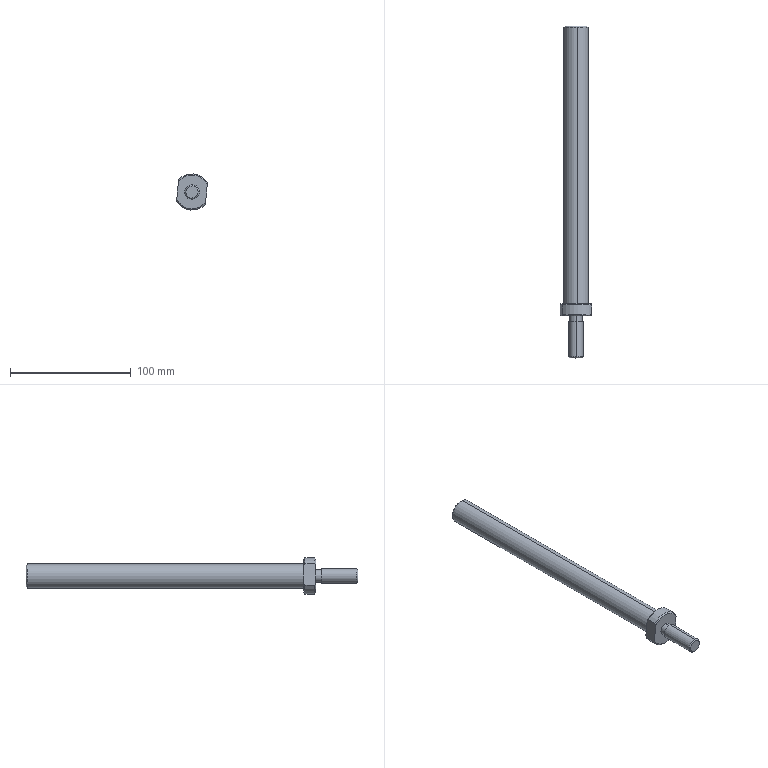Component | SolidWorks | 8TC-A15004-80-16A-3 | 1 solid | 26 faces | box 25.76 x 275 x 30 mm | volume 82271 mm3 | cone 10 | cylinder 9 | plane 7 | commonest cylinder face diameters 30 x3 20 x2 10 x2 12 x2 | material #45
build123d program:
from build123d import *

# Parameters (mm, degrees)
CHAMFER1_SIZE       = 1
SKETCH2_OUTSIDE_W   = 87.65
SKETCH2_OUTSIDE_H   = 87.65
SKETCH2_OUTSIDE_W_2 = 30
SKETCH2_OUTSIDE_H_2 = 24
CUT_EXTRUDE2_DEPTH  = 276.817


with BuildPart() as part:
    # Sketch1 → Revolve3 (revolve)
    with BuildSketch(Plane(origin=(0, 0, 0), x_dir=(1, 0, 0), z_dir=(0, 1, 0)), mode=Mode.PRIVATE) as revolve3_sk:
        Polygon((0, 0), (0, 6), (30, 6), (30, 5), (35, 5), (35, 15), (45, 15), (45, 10), (275, 10), (275, 0), align=None)
    revolve(revolve3_sk.sketch.rotate(Axis((0, 0, 0), (1, 0, 0)), 180), axis=Axis((0, 0, 0), (1, 0, 0)))

    # Chamfer1
    chamfer1_edges = [part.edges().sort_by_distance(p)[0] for p in [
        (0, 0, -6),
        (275, 0, -10),
        (45, 0, -15),
        (35, 0, -15),
    ]]
    chamfer(chamfer1_edges, length=CHAMFER1_SIZE)

    # Sketch2 outside → Cut-Extrude2 (cut, through all)
    with BuildSketch(Plane(origin=(275, 0, 0), x_dir=(0, 0, -1), z_dir=(1, 0, 0))):
        Rectangle(SKETCH2_OUTSIDE_W, SKETCH2_OUTSIDE_H)
        Rectangle(SKETCH2_OUTSIDE_W_2, SKETCH2_OUTSIDE_H_2, mode=Mode.SUBTRACT)
    extrude(amount=-CUT_EXTRUDE2_DEPTH, mode=Mode.SUBTRACT)


solid = part.part

# Placed as in the assembly
solid = solid.moved(Location((40, -42.5, -750), (-180, -6.034, -90)))
STEP:
#1=CARTESIAN_POINT('',(1.554,-1.673,-29.723));
#2=VERTEX_POINT('',#1);
#3=CARTESIAN_POINT('',(1.595,-1.673,-29.332));
#4=VERTEX_POINT('',#3);
#5=CARTESIAN_POINT('',(1.575,-1.673,-29.528));
#6=DIRECTION('',(0.,-1.,0.));
#7=DIRECTION('',(0.1051,0.,0.9945));
#8=AXIS2_PLACEMENT_3D('',#5,#6,#7);
#9=CIRCLE('',#8,0.1969);
#10=EDGE_CURVE('',#2,#4,#9,.T.);
#11=ORIENTED_EDGE('',*,*,#10,.F.);
#12=CARTESIAN_POINT('',(1.55,-1.634,-29.762));
#13=VERTEX_POINT('',#12);
#14=CARTESIAN_POINT('',(1.554,-1.673,-29.723));
#15=DIRECTION('',(-0.07432,0.7071,-0.7032));
#16=VECTOR('',#15,39.37);
#17=LINE('',#14,#16);
#18=EDGE_CURVE('',#2,#13,#17,.T.);
#19=ORIENTED_EDGE('',*,*,#18,.T.);
#20=CARTESIAN_POINT('',(1.6,-1.634,-29.293));
#21=VERTEX_POINT('',#20);
#22=CARTESIAN_POINT('',(1.575,-1.634,-29.528));
#23=DIRECTION('',(0.,1.,0.));
#24=DIRECTION('',(0.1051,0.,0.9945));
#25=AXIS2_PLACEMENT_3D('',#22,#23,#24);
#26=CIRCLE('',#25,0.2362);
#27=EDGE_CURVE('',#21,#13,#26,.T.);
#28=ORIENTED_EDGE('',*,*,#27,.F.);
#29=CARTESIAN_POINT('',(1.595,-1.673,-29.332));
#30=DIRECTION('',(0.07432,0.7071,0.7032));
#31=VECTOR('',#30,39.37);
#32=LINE('',#29,#31);
#33=EDGE_CURVE('',#4,#21,#32,.T.);
#34=ORIENTED_EDGE('',*,*,#33,.F.);
#35=EDGE_LOOP('',(#11,#19,#28,#34));
#36=FACE_OUTER_BOUND('',#35,.T.);
#37=CARTESIAN_POINT('',(1.575,-1.673,-29.528));
#38=DIRECTION('',(0.,1.,0.));
#39=DIRECTION('',(0.1051,0.,0.9945));
#40=AXIS2_PLACEMENT_3D('',#37,#38,#39);
#41=CONICAL_SURFACE('',#40,0.1969,0.7854);
#42=ADVANCED_FACE('',(#36),#41,.T.);
#43=CARTESIAN_POINT('',(1.612,9.154,-29.175));
#44=VERTEX_POINT('',#43);
#45=CARTESIAN_POINT('',(1.538,9.154,-29.88));
#46=VERTEX_POINT('',#45);
#47=CARTESIAN_POINT('',(1.575,9.154,-29.528));
#48=DIRECTION('',(0.,1.,0.));
#49=DIRECTION('',(-0.1051,0.,-0.9945));
#50=AXIS2_PLACEMENT_3D('',#47,#48,#49);
#51=CIRCLE('',#50,0.3543);
#52=EDGE_CURVE('',#44,#46,#51,.T.);
#53=ORIENTED_EDGE('',*,*,#52,.F.);
#54=CARTESIAN_POINT('',(1.616,9.114,-29.136));
#55=VERTEX_POINT('',#54);
#56=CARTESIAN_POINT('',(1.616,9.114,-29.136));
#57=DIRECTION('',(0.07432,-0.7071,0.7032));
#58=VECTOR('',#57,39.37);
#59=LINE('',#56,#58);
#60=EDGE_CURVE('',#44,#55,#59,.T.);
#61=ORIENTED_EDGE('',*,*,#60,.T.);
#62=CARTESIAN_POINT('',(1.533,9.114,-29.919));
#63=VERTEX_POINT('',#62);
#64=CARTESIAN_POINT('',(1.575,9.114,-29.528));
#65=DIRECTION('',(0.,-1.,0.));
#66=DIRECTION('',(-0.1051,0.,-0.9945));
#67=AXIS2_PLACEMENT_3D('',#64,#65,#66);
#68=CIRCLE('',#67,0.3937);
#69=EDGE_CURVE('',#63,#55,#68,.T.);
#70=ORIENTED_EDGE('',*,*,#69,.F.);
#71=CARTESIAN_POINT('',(1.533,9.114,-29.919));
#72=DIRECTION('',(-0.07432,-0.7071,-0.7032));
#73=VECTOR('',#72,39.37);
#74=LINE('',#71,#73);
#75=EDGE_CURVE('',#46,#63,#74,.T.);
#76=ORIENTED_EDGE('',*,*,#75,.F.);
#77=EDGE_LOOP('',(#53,#61,#70,#76));
#78=FACE_OUTER_BOUND('',#77,.T.);
#79=CARTESIAN_POINT('',(1.575,9.114,-29.528));
#80=DIRECTION('',(0.,-1.,0.));
#81=DIRECTION('',(-0.1051,0.,-0.9945));
#82=AXIS2_PLACEMENT_3D('',#79,#80,#81);
#83=CONICAL_SURFACE('',#82,0.3937,0.7854);
#84=ADVANCED_FACE('',(#78),#83,.T.);
#85=ORIENTED_EDGE('',*,*,#69,.T.);
#86=CARTESIAN_POINT('',(1.616,0.09843,-29.136));
#87=VERTEX_POINT('',#86);
#88=CARTESIAN_POINT('',(1.616,-1.673,-29.136));
#89=DIRECTION('',(0.,-1.,0.));
#90=VECTOR('',#89,39.37);
#91=LINE('',#88,#90);
#92=EDGE_CURVE('',#55,#87,#91,.T.);
#93=ORIENTED_EDGE('',*,*,#92,.T.);
#94=CARTESIAN_POINT('',(1.533,0.09843,-29.919));
#95=VERTEX_POINT('',#94);
#96=CARTESIAN_POINT('',(1.575,0.09843,-29.528));
#97=DIRECTION('',(0.,-1.,0.));
#98=DIRECTION('',(-0.1051,0.,-0.9945));
#99=AXIS2_PLACEMENT_3D('',#96,#97,#98);
#100=CIRCLE('',#99,0.3937);
#101=EDGE_CURVE('',#95,#87,#100,.T.);
#102=ORIENTED_EDGE('',*,*,#101,.F.);
#103=CARTESIAN_POINT('',(1.533,-1.673,-29.919));
#104=DIRECTION('',(0.,-1.,0.));
#105=VECTOR('',#104,39.37);
#106=LINE('',#103,#105);
#107=EDGE_CURVE('',#63,#95,#106,.T.);
#108=ORIENTED_EDGE('',*,*,#107,.F.);
#109=EDGE_LOOP('',(#85,#93,#102,#108));
#110=FACE_OUTER_BOUND('',#109,.T.);
#111=CARTESIAN_POINT('',(1.575,-1.673,-29.528));
#112=DIRECTION('',(0.,-1.,0.));
#113=DIRECTION('',(-0.1051,0.,-0.9945));
#114=AXIS2_PLACEMENT_3D('',#111,#112,#113);
#115=CYLINDRICAL_SURFACE('',#114,0.3937);
#116=ADVANCED_FACE('',(#110),#115,.T.);
#117=CARTESIAN_POINT('',(1.554,-0.2953,-29.723));
#118=VERTEX_POINT('',#117);
#119=CARTESIAN_POINT('',(1.595,-0.2953,-29.332));
#120=VERTEX_POINT('',#119);
#121=CARTESIAN_POINT('',(1.575,-0.2953,-29.528));
#122=DIRECTION('',(0.,-1.,0.));
#123=DIRECTION('',(-0.1051,0.,-0.9945));
#124=AXIS2_PLACEMENT_3D('',#121,#122,#123);
#125=CIRCLE('',#124,0.1969);
#126=EDGE_CURVE('',#118,#120,#125,.T.);
#127=ORIENTED_EDGE('',*,*,#126,.T.);
#128=CARTESIAN_POINT('',(1.595,-0.4921,-29.332));
#129=VERTEX_POINT('',#128);
#130=CARTESIAN_POINT('',(1.595,-1.673,-29.332));
#131=DIRECTION('',(0.,-1.,0.));
#132=VECTOR('',#131,39.37);
#133=LINE('',#130,#132);
#134=EDGE_CURVE('',#120,#129,#133,.T.);
#135=ORIENTED_EDGE('',*,*,#134,.T.);
#136=CARTESIAN_POINT('',(1.554,-0.4921,-29.723));
#137=VERTEX_POINT('',#136);
#138=CARTESIAN_POINT('',(1.575,-0.4921,-29.528));
#139=DIRECTION('',(0.,-1.,0.));
#140=DIRECTION('',(-0.1051,0.,-0.9945));
#141=AXIS2_PLACEMENT_3D('',#138,#139,#140);
#142=CIRCLE('',#141,0.1969);
#143=EDGE_CURVE('',#137,#129,#142,.T.);
#144=ORIENTED_EDGE('',*,*,#143,.F.);
#145=CARTESIAN_POINT('',(1.554,-1.673,-29.723));
#146=DIRECTION('',(0.,-1.,0.));
#147=VECTOR('',#146,39.37);
#148=LINE('',#145,#147);
#149=EDGE_CURVE('',#118,#137,#148,.T.);
#150=ORIENTED_EDGE('',*,*,#149,.F.);
#151=EDGE_LOOP('',(#127,#135,#144,#150));
#152=FACE_OUTER_BOUND('',#151,.T.);
#153=CARTESIAN_POINT('',(1.575,-1.673,-29.528));
#154=DIRECTION('',(0.,-1.,0.));
#155=DIRECTION('',(-0.1051,0.,-0.9945));
#156=AXIS2_PLACEMENT_3D('',#153,#154,#155);
#157=CYLINDRICAL_SURFACE('',#156,0.1969);
#158=ADVANCED_FACE('',(#152),#157,.T.);
#159=CARTESIAN_POINT('',(1.55,-0.4921,-29.762));
#160=VERTEX_POINT('',#159);
#161=CARTESIAN_POINT('',(1.6,-0.4921,-29.293));
#162=VERTEX_POINT('',#161);
#163=CARTESIAN_POINT('',(1.575,-0.4921,-29.528));
#164=DIRECTION('',(0.,-1.,0.));
#165=DIRECTION('',(-0.1051,0.,-0.9945));
#166=AXIS2_PLACEMENT_3D('',#163,#164,#165);
#167=CIRCLE('',#166,0.2362);
#168=EDGE_CURVE('',#160,#162,#167,.T.);
#169=ORIENTED_EDGE('',*,*,#168,.T.);
#170=CARTESIAN_POINT('',(1.6,-1.673,-29.293));
#171=DIRECTION('',(0.,-1.,0.));
#172=VECTOR('',#171,39.37);
#173=LINE('',#170,#172);
#174=EDGE_CURVE('',#162,#21,#173,.T.);
#175=ORIENTED_EDGE('',*,*,#174,.T.);
#176=ORIENTED_EDGE('',*,*,#27,.T.);
#177=CARTESIAN_POINT('',(1.55,-1.673,-29.762));
#178=DIRECTION('',(0.,-1.,0.));
#179=VECTOR('',#178,39.37);
#180=LINE('',#177,#179);
#181=EDGE_CURVE('',#160,#13,#180,.T.);
#182=ORIENTED_EDGE('',*,*,#181,.F.);
#183=EDGE_LOOP('',(#169,#175,#176,#182));
#184=FACE_OUTER_BOUND('',#183,.T.);
#185=CARTESIAN_POINT('',(1.575,-1.673,-29.528));
#186=DIRECTION('',(0.,-1.,0.));
#187=DIRECTION('',(-0.1051,0.,-0.9945));
#188=AXIS2_PLACEMENT_3D('',#185,#186,#187);
#189=CYLINDRICAL_SURFACE('',#188,0.2362);
#190=ADVANCED_FACE('',(#184),#189,.T.);
#191=CARTESIAN_POINT('',(1.633,-0.2953,-28.979));
#192=VERTEX_POINT('',#191);
#193=CARTESIAN_POINT('',(1.135,-0.2953,-29.196));
#194=VERTEX_POINT('',#193);
#195=CARTESIAN_POINT('',(1.575,-0.2953,-29.528));
#196=DIRECTION('',(0.,-1.,0.));
#197=DIRECTION('',(0.1051,0.,0.9945));
#198=AXIS2_PLACEMENT_3D('',#195,#196,#197);
#199=CIRCLE('',#198,0.5512);
#200=EDGE_CURVE('',#192,#194,#199,.T.);
#201=ORIENTED_EDGE('',*,*,#200,.F.);
#202=CARTESIAN_POINT('',(1.637,-0.2559,-28.94));
#203=VERTEX_POINT('',#202);
#204=CARTESIAN_POINT('',(1.633,-0.2953,-28.979));
#205=DIRECTION('',(0.07432,0.7071,0.7032));
#206=VECTOR('',#205,39.37);
#207=LINE('',#204,#206);
#208=EDGE_CURVE('',#192,#203,#207,.T.);
#209=ORIENTED_EDGE('',*,*,#208,.T.);
#210=CARTESIAN_POINT('',(1.142,-0.2559,-29.126));
#211=VERTEX_POINT('',#210);
#212=CARTESIAN_POINT('',(1.575,-0.2559,-29.528));
#213=DIRECTION('',(0.,1.,0.));
#214=DIRECTION('',(0.1051,0.,0.9945));
#215=AXIS2_PLACEMENT_3D('',#212,#213,#214);
#216=CIRCLE('',#215,0.5906);
#217=EDGE_CURVE('',#211,#203,#216,.T.);
#218=ORIENTED_EDGE('',*,*,#217,.F.);
#219=CARTESIAN_POINT('',(1.142,-0.2559,-29.126));
#220=CARTESIAN_POINT('',(1.14,-0.2698,-29.149));
#221=CARTESIAN_POINT('',(1.137,-0.283,-29.172));
#222=CARTESIAN_POINT('',(1.135,-0.2953,-29.196));
#223=B_SPLINE_CURVE_WITH_KNOTS('',3,(#219,#220,#221,#222),.UNSPECIFIED.,.F.,.F.,(4,4),(0.02828,0.03033),.UNSPECIFIED.);
#224=EDGE_CURVE('',#211,#194,#223,.T.);
#225=ORIENTED_EDGE('',*,*,#224,.T.);
#226=EDGE_LOOP('',(#201,#209,#218,#225));
#227=FACE_OUTER_BOUND('',#226,.T.);
#228=CARTESIAN_POINT('',(1.575,-0.2953,-29.528));
#229=DIRECTION('',(0.,1.,0.));
#230=DIRECTION('',(0.1051,0.,0.9945));
#231=AXIS2_PLACEMENT_3D('',#228,#229,#230);
#232=CONICAL_SURFACE('',#231,0.5512,0.7854);
#233=ADVANCED_FACE('',(#227),#232,.T.);
#234=CARTESIAN_POINT('',(1.517,0.09843,-30.076));
#235=VERTEX_POINT('',#234);
#236=CARTESIAN_POINT('',(1.075,0.09843,-29.76));
#237=VERTEX_POINT('',#236);
#238=CARTESIAN_POINT('',(1.575,0.09843,-29.528));
#239=DIRECTION('',(0.,1.,0.));
#240=DIRECTION('',(-0.1051,0.,-0.9945));
#241=AXIS2_PLACEMENT_3D('',#238,#239,#240);
#242=CIRCLE('',#241,0.5512);
#243=EDGE_CURVE('',#235,#237,#242,.T.);
#244=ORIENTED_EDGE('',*,*,#243,.F.);
#245=CARTESIAN_POINT('',(1.513,0.05906,-30.115));
#246=VERTEX_POINT('',#245);
#247=CARTESIAN_POINT('',(1.513,0.05906,-30.115));
#248=DIRECTION('',(-0.07432,-0.7071,-0.7032));
#249=VECTOR('',#248,39.37);
#250=LINE('',#247,#249);
#251=EDGE_CURVE('',#235,#246,#250,.T.);
#252=ORIENTED_EDGE('',*,*,#251,.T.);
#253=CARTESIAN_POINT('',(1.068,0.05906,-29.83));
#254=VERTEX_POINT('',#253);
#255=CARTESIAN_POINT('',(1.575,0.05906,-29.528));
#256=DIRECTION('',(0.,-1.,0.));
#257=DIRECTION('',(-0.1051,0.,-0.9945));
#258=AXIS2_PLACEMENT_3D('',#255,#256,#257);
#259=CIRCLE('',#258,0.5906);
#260=EDGE_CURVE('',#254,#246,#259,.T.);
#261=ORIENTED_EDGE('',*,*,#260,.F.);
#262=CARTESIAN_POINT('',(1.068,0.05906,-29.83));
#263=CARTESIAN_POINT('',(1.07,0.07292,-29.807));
#264=CARTESIAN_POINT('',(1.073,0.08613,-29.784));
#265=CARTESIAN_POINT('',(1.075,0.09843,-29.76));
#266=B_SPLINE_CURVE_WITH_KNOTS('',3,(#262,#263,#264,#265),.UNSPECIFIED.,.F.,.F.,(4,4),(0.02828,0.03033),.UNSPECIFIED.);
#267=EDGE_CURVE('',#254,#237,#266,.T.);
#268=ORIENTED_EDGE('',*,*,#267,.T.);
#269=EDGE_LOOP('',(#244,#252,#261,#268));
#270=FACE_OUTER_BOUND('',#269,.T.);
#271=CARTESIAN_POINT('',(1.575,0.05906,-29.528));
#272=DIRECTION('',(0.,-1.,0.));
#273=DIRECTION('',(-0.1051,0.,-0.9945));
#274=AXIS2_PLACEMENT_3D('',#271,#272,#273);
#275=CONICAL_SURFACE('',#274,0.5906,0.7854);
#276=ADVANCED_FACE('',(#270),#275,.T.);
#277=ORIENTED_EDGE('',*,*,#260,.T.);
#278=CARTESIAN_POINT('',(1.513,-0.2559,-30.115));
#279=VERTEX_POINT('',#278);
#280=CARTESIAN_POINT('',(1.513,-1.673,-30.115));
#281=DIRECTION('',(0.,-1.,0.));
#282=VECTOR('',#281,39.37);
#283=LINE('',#280,#282);
#284=EDGE_CURVE('',#246,#279,#283,.T.);
#285=ORIENTED_EDGE('',*,*,#284,.T.);
#286=CARTESIAN_POINT('',(1.068,-0.2559,-29.83));
#287=VERTEX_POINT('',#286);
#288=CARTESIAN_POINT('',(1.575,-0.2559,-29.528));
#289=DIRECTION('',(0.,1.,0.));
#290=DIRECTION('',(0.1051,0.,0.9945));
#291=AXIS2_PLACEMENT_3D('',#288,#289,#290);
#292=CIRCLE('',#291,0.5906);
#293=EDGE_CURVE('',#279,#287,#292,.T.);
#294=ORIENTED_EDGE('',*,*,#293,.T.);
#295=CARTESIAN_POINT('',(1.068,-1.673,-29.83));
#296=DIRECTION('',(0.,-1.,0.));
#297=VECTOR('',#296,39.37);
#298=LINE('',#295,#297);
#299=EDGE_CURVE('',#254,#287,#298,.T.);
#300=ORIENTED_EDGE('',*,*,#299,.F.);
#301=EDGE_LOOP('',(#277,#285,#294,#300));
#302=FACE_OUTER_BOUND('',#301,.T.);
#303=CARTESIAN_POINT('',(1.575,-1.673,-29.528));
#304=DIRECTION('',(0.,-1.,0.));
#305=DIRECTION('',(-0.1051,0.,-0.9945));
#306=AXIS2_PLACEMENT_3D('',#303,#304,#305);
#307=CYLINDRICAL_SURFACE('',#306,0.5906);
#308=ADVANCED_FACE('',(#302),#307,.T.);
#309=ORIENTED_EDGE('',*,*,#126,.F.);
#310=CARTESIAN_POINT('',(1.575,-0.2953,-29.528));
#311=DIRECTION('',(0.,-1.,0.));
#312=DIRECTION('',(-0.1051,0.,-0.9945));
#313=AXIS2_PLACEMENT_3D('',#310,#311,#312);
#314=CIRCLE('',#313,0.1969);
#315=EDGE_CURVE('',#120,#118,#314,.T.);
#316=ORIENTED_EDGE('',*,*,#315,.F.);
#317=EDGE_LOOP('',(#309,#316));
#318=FACE_BOUND('',#317,.T.);
#319=CARTESIAN_POINT('',(1.075,-0.2953,-29.76));
#320=VERTEX_POINT('',#319);
#321=CARTESIAN_POINT('',(1.126,-0.2953,-29.282));
#322=DIRECTION('',(0.1051,0.,0.9945));
#323=VECTOR('',#322,39.37);
#324=LINE('',#321,#323);
#325=EDGE_CURVE('',#320,#194,#324,.T.);
#326=ORIENTED_EDGE('',*,*,#325,.F.);
#327=CARTESIAN_POINT('',(2.015,-0.2953,-29.86));
#328=VERTEX_POINT('',#327);
#329=CARTESIAN_POINT('',(1.575,-0.2953,-29.528));
#330=DIRECTION('',(0.,-1.,0.));
#331=DIRECTION('',(0.1051,0.,0.9945));
#332=AXIS2_PLACEMENT_3D('',#329,#330,#331);
#333=CIRCLE('',#332,0.5512);
#334=EDGE_CURVE('',#320,#328,#333,.T.);
#335=ORIENTED_EDGE('',*,*,#334,.T.);
#336=CARTESIAN_POINT('',(2.074,-0.2953,-29.295));
#337=VERTEX_POINT('',#336);
#338=CARTESIAN_POINT('',(2.065,-0.2953,-29.381));
#339=DIRECTION('',(-0.1051,0.,-0.9945));
#340=VECTOR('',#339,39.37);
#341=LINE('',#338,#340);
#342=EDGE_CURVE('',#337,#328,#341,.T.);
#343=ORIENTED_EDGE('',*,*,#342,.F.);
#344=CARTESIAN_POINT('',(1.575,-0.2953,-29.528));
#345=DIRECTION('',(0.,-1.,0.));
#346=DIRECTION('',(0.1051,0.,0.9945));
#347=AXIS2_PLACEMENT_3D('',#344,#345,#346);
#348=CIRCLE('',#347,0.5512);
#349=EDGE_CURVE('',#337,#192,#348,.T.);
#350=ORIENTED_EDGE('',*,*,#349,.T.);
#351=ORIENTED_EDGE('',*,*,#200,.T.);
#352=EDGE_LOOP('',(#326,#335,#343,#350,#351));
#353=FACE_OUTER_BOUND('',#352,.T.);
#354=CARTESIAN_POINT('',(1.595,-0.2953,-29.332));
#355=DIRECTION('',(0.,1.,0.));
#356=DIRECTION('',(0.1051,0.,0.9945));
#357=AXIS2_PLACEMENT_3D('',#354,#355,#356);
#358=PLANE('',#357);
#359=ADVANCED_FACE('',(#318,#353),#358,.F.);
#360=CARTESIAN_POINT('',(2.082,0.05906,-29.225));
#361=VERTEX_POINT('',#360);
#362=CARTESIAN_POINT('',(1.142,0.05906,-29.126));
#363=VERTEX_POINT('',#362);
#364=CARTESIAN_POINT('',(1.575,0.05906,-29.528));
#365=DIRECTION('',(0.,-1.,0.));
#366=DIRECTION('',(-0.1051,0.,-0.9945));
#367=AXIS2_PLACEMENT_3D('',#364,#365,#366);
#368=CIRCLE('',#367,0.5906);
#369=EDGE_CURVE('',#361,#363,#368,.T.);
#370=ORIENTED_EDGE('',*,*,#369,.T.);
#371=CARTESIAN_POINT('',(1.142,-1.673,-29.126));
#372=DIRECTION('',(0.,1.,0.));
#373=VECTOR('',#372,39.37);
#374=LINE('',#371,#373);
#375=EDGE_CURVE('',#211,#363,#374,.T.);
#376=ORIENTED_EDGE('',*,*,#375,.F.);
#377=ORIENTED_EDGE('',*,*,#217,.T.);
#378=CARTESIAN_POINT('',(2.082,-0.2559,-29.225));
#379=VERTEX_POINT('',#378);
#380=CARTESIAN_POINT('',(1.575,-0.2559,-29.528));
#381=DIRECTION('',(0.,1.,0.));
#382=DIRECTION('',(0.1051,0.,0.9945));
#383=AXIS2_PLACEMENT_3D('',#380,#381,#382);
#384=CIRCLE('',#383,0.5906);
#385=EDGE_CURVE('',#203,#379,#384,.T.);
#386=ORIENTED_EDGE('',*,*,#385,.T.);
#387=CARTESIAN_POINT('',(2.082,-1.673,-29.225));
#388=DIRECTION('',(0.,-1.,0.));
#389=VECTOR('',#388,39.37);
#390=LINE('',#387,#389);
#391=EDGE_CURVE('',#361,#379,#390,.T.);
#392=ORIENTED_EDGE('',*,*,#391,.F.);
#393=EDGE_LOOP('',(#370,#376,#377,#386,#392));
#394=FACE_OUTER_BOUND('',#393,.T.);
#395=CARTESIAN_POINT('',(1.575,-1.673,-29.528));
#396=DIRECTION('',(0.,-1.,0.));
#397=DIRECTION('',(-0.1051,0.,-0.9945));
#398=AXIS2_PLACEMENT_3D('',#395,#396,#397);
#399=CYLINDRICAL_SURFACE('',#398,0.5906);
#400=ADVANCED_FACE('',(#394),#399,.T.);
#401=ORIENTED_EDGE('',*,*,#284,.F.);
#402=CARTESIAN_POINT('',(2.007,0.05906,-29.93));
#403=VERTEX_POINT('',#402);
#404=CARTESIAN_POINT('',(1.575,0.05906,-29.528));
#405=DIRECTION('',(0.,-1.,0.));
#406=DIRECTION('',(-0.1051,0.,-0.9945));
#407=AXIS2_PLACEMENT_3D('',#404,#405,#406);
#408=CIRCLE('',#407,0.5906);
#409=EDGE_CURVE('',#246,#403,#408,.T.);
#410=ORIENTED_EDGE('',*,*,#409,.T.);
#411=CARTESIAN_POINT('',(2.007,-0.2559,-29.93));
#412=VERTEX_POINT('',#411);
#413=CARTESIAN_POINT('',(2.007,-1.673,-29.93));
#414=DIRECTION('',(0.,1.,0.));
#415=VECTOR('',#414,39.37);
#416=LINE('',#413,#415);
#417=EDGE_CURVE('',#412,#403,#416,.T.);
#418=ORIENTED_EDGE('',*,*,#417,.F.);
#419=CARTESIAN_POINT('',(1.575,-0.2559,-29.528));
#420=DIRECTION('',(0.,1.,0.));
#421=DIRECTION('',(0.1051,0.,0.9945));
#422=AXIS2_PLACEMENT_3D('',#419,#420,#421);
#423=CIRCLE('',#422,0.5906);
#424=EDGE_CURVE('',#412,#279,#423,.T.);
#425=ORIENTED_EDGE('',*,*,#424,.T.);
#426=EDGE_LOOP('',(#401,#410,#418,#425));
#427=FACE_OUTER_BOUND('',#426,.T.);
#428=CARTESIAN_POINT('',(1.575,-1.673,-29.528));
#429=DIRECTION('',(0.,-1.,0.));
#430=DIRECTION('',(-0.1051,0.,-0.9945));
#431=AXIS2_PLACEMENT_3D('',#428,#429,#430);
#432=CYLINDRICAL_SURFACE('',#431,0.5906);
#433=ADVANCED_FACE('',(#427),#432,.T.);
#434=ORIENTED_EDGE('',*,*,#101,.T.);
#435=CARTESIAN_POINT('',(1.575,0.09843,-29.528));
#436=DIRECTION('',(0.,-1.,0.));
#437=DIRECTION('',(-0.1051,0.,-0.9945));
#438=AXIS2_PLACEMENT_3D('',#435,#436,#437);
#439=CIRCLE('',#438,0.3937);
#440=EDGE_CURVE('',#87,#95,#439,.T.);
#441=ORIENTED_EDGE('',*,*,#440,.T.);
#442=EDGE_LOOP('',(#434,#441));
#443=FACE_BOUND('',#442,.T.);
#444=CARTESIAN_POINT('',(1.135,0.09843,-29.196));
#445=VERTEX_POINT('',#444);
#446=CARTESIAN_POINT('',(1.167,0.09843,-28.891));
#447=DIRECTION('',(-0.1051,0.,-0.9945));
#448=VECTOR('',#447,39.37);
#449=LINE('',#446,#448);
#450=EDGE_CURVE('',#445,#237,#449,.T.);
#451=ORIENTED_EDGE('',*,*,#450,.F.);
#452=CARTESIAN_POINT('',(2.074,0.09843,-29.295));
#453=VERTEX_POINT('',#452);
#454=CARTESIAN_POINT('',(1.575,0.09843,-29.528));
#455=DIRECTION('',(0.,1.,0.));
#456=DIRECTION('',(-0.1051,0.,-0.9945));
#457=AXIS2_PLACEMENT_3D('',#454,#455,#456);
#458=CIRCLE('',#457,0.5512);
#459=EDGE_CURVE('',#445,#453,#458,.T.);
#460=ORIENTED_EDGE('',*,*,#459,.T.);
#461=CARTESIAN_POINT('',(2.015,0.09843,-29.86));
#462=VERTEX_POINT('',#461);
#463=CARTESIAN_POINT('',(2.107,0.09843,-28.99));
#464=DIRECTION('',(0.1051,0.,0.9945));
#465=VECTOR('',#464,39.37);
#466=LINE('',#463,#465);
#467=EDGE_CURVE('',#462,#453,#466,.T.);
#468=ORIENTED_EDGE('',*,*,#467,.F.);
#469=CARTESIAN_POINT('',(1.575,0.09843,-29.528));
#470=DIRECTION('',(0.,1.,0.));
#471=DIRECTION('',(-0.1051,0.,-0.9945));
#472=AXIS2_PLACEMENT_3D('',#469,#470,#471);
#473=CIRCLE('',#472,0.5512);
#474=EDGE_CURVE('',#462,#235,#473,.T.);
#475=ORIENTED_EDGE('',*,*,#474,.T.);
#476=ORIENTED_EDGE('',*,*,#243,.T.);
#477=EDGE_LOOP('',(#451,#460,#468,#475,#476));
#478=FACE_OUTER_BOUND('',#477,.T.);
#479=CARTESIAN_POINT('',(1.637,0.09843,-28.94));
#480=DIRECTION('',(0.,-1.,0.));
#481=DIRECTION('',(-0.1051,0.,-0.9945));
#482=AXIS2_PLACEMENT_3D('',#479,#480,#481);
#483=PLANE('',#482);
#484=ADVANCED_FACE('',(#443,#478),#483,.F.);
#485=ORIENTED_EDGE('',*,*,#251,.F.);
#486=ORIENTED_EDGE('',*,*,#474,.F.);
#487=CARTESIAN_POINT('',(2.015,0.09843,-29.86));
#488=CARTESIAN_POINT('',(2.012,0.0861,-29.883));
#489=CARTESIAN_POINT('',(2.01,0.0729,-29.907));
#490=CARTESIAN_POINT('',(2.007,0.05906,-29.93));
#491=B_SPLINE_CURVE_WITH_KNOTS('',3,(#487,#488,#489,#490),.UNSPECIFIED.,.F.,.F.,(4,4),(0.04546,0.04753),.UNSPECIFIED.);
#492=EDGE_CURVE('',#462,#403,#491,.T.);
#493=ORIENTED_EDGE('',*,*,#492,.T.);
#494=ORIENTED_EDGE('',*,*,#409,.F.);
#495=EDGE_LOOP('',(#485,#486,#493,#494));
#496=FACE_OUTER_BOUND('',#495,.T.);
#497=CARTESIAN_POINT('',(1.575,0.05906,-29.528));
#498=DIRECTION('',(0.,-1.,0.));
#499=DIRECTION('',(-0.1051,0.,-0.9945));
#500=AXIS2_PLACEMENT_3D('',#497,#498,#499);
#501=CONICAL_SURFACE('',#500,0.5906,0.7854);
#502=ADVANCED_FACE('',(#496),#501,.T.);
#503=ORIENTED_EDGE('',*,*,#459,.F.);
#504=CARTESIAN_POINT('',(1.135,0.09843,-29.196));
#505=CARTESIAN_POINT('',(1.137,0.0861,-29.172));
#506=CARTESIAN_POINT('',(1.14,0.0729,-29.148));
#507=CARTESIAN_POINT('',(1.142,0.05906,-29.126));
#508=B_SPLINE_CURVE_WITH_KNOTS('',3,(#504,#505,#506,#507),.UNSPECIFIED.,.F.,.F.,(4,4),(0.04546,0.04753),.UNSPECIFIED.);
#509=EDGE_CURVE('',#445,#363,#508,.T.);
#510=ORIENTED_EDGE('',*,*,#509,.T.);
#511=ORIENTED_EDGE('',*,*,#369,.F.);
#512=CARTESIAN_POINT('',(2.082,0.05906,-29.225));
#513=CARTESIAN_POINT('',(2.079,0.07292,-29.248));
#514=CARTESIAN_POINT('',(2.077,0.08613,-29.271));
#515=CARTESIAN_POINT('',(2.074,0.09843,-29.295));
#516=B_SPLINE_CURVE_WITH_KNOTS('',3,(#512,#513,#514,#515),.UNSPECIFIED.,.F.,.F.,(4,4),(0.02828,0.03033),.UNSPECIFIED.);
#517=EDGE_CURVE('',#361,#453,#516,.T.);
#518=ORIENTED_EDGE('',*,*,#517,.T.);
#519=EDGE_LOOP('',(#503,#510,#511,#518));
#520=FACE_OUTER_BOUND('',#519,.T.);
#521=CARTESIAN_POINT('',(1.575,0.05906,-29.528));
#522=DIRECTION('',(0.,-1.,0.));
#523=DIRECTION('',(-0.1051,0.,-0.9945));
#524=AXIS2_PLACEMENT_3D('',#521,#522,#523);
#525=CONICAL_SURFACE('',#524,0.5906,0.7854);
#526=ADVANCED_FACE('',(#520),#525,.T.);
#527=ORIENTED_EDGE('',*,*,#208,.F.);
#528=ORIENTED_EDGE('',*,*,#349,.F.);
#529=CARTESIAN_POINT('',(2.074,-0.2953,-29.295));
#530=CARTESIAN_POINT('',(2.077,-0.2829,-29.271));
#531=CARTESIAN_POINT('',(2.079,-0.2697,-29.248));
#532=CARTESIAN_POINT('',(2.082,-0.2559,-29.225));
#533=B_SPLINE_CURVE_WITH_KNOTS('',3,(#529,#530,#531,#532),.UNSPECIFIED.,.F.,.F.,(4,4),(0.04546,0.04753),.UNSPECIFIED.);
#534=EDGE_CURVE('',#337,#379,#533,.T.);
#535=ORIENTED_EDGE('',*,*,#534,.T.);
#536=ORIENTED_EDGE('',*,*,#385,.F.);
#537=EDGE_LOOP('',(#527,#528,#535,#536));
#538=FACE_OUTER_BOUND('',#537,.T.);
#539=CARTESIAN_POINT('',(1.575,-0.2953,-29.528));
#540=DIRECTION('',(0.,1.,0.));
#541=DIRECTION('',(0.1051,0.,0.9945));
#542=AXIS2_PLACEMENT_3D('',#539,#540,#541);
#543=CONICAL_SURFACE('',#542,0.5512,0.7854);
#544=ADVANCED_FACE('',(#538),#543,.T.);
#545=ORIENTED_EDGE('',*,*,#334,.F.);
#546=CARTESIAN_POINT('',(1.075,-0.2953,-29.76));
#547=CARTESIAN_POINT('',(1.073,-0.2829,-29.784));
#548=CARTESIAN_POINT('',(1.07,-0.2697,-29.807));
#549=CARTESIAN_POINT('',(1.068,-0.2559,-29.83));
#550=B_SPLINE_CURVE_WITH_KNOTS('',3,(#546,#547,#548,#549),.UNSPECIFIED.,.F.,.F.,(4,4),(0.04546,0.04753),.UNSPECIFIED.);
#551=EDGE_CURVE('',#320,#287,#550,.T.);
#552=ORIENTED_EDGE('',*,*,#551,.T.);
#553=ORIENTED_EDGE('',*,*,#293,.F.);
#554=ORIENTED_EDGE('',*,*,#424,.F.);
#555=CARTESIAN_POINT('',(2.007,-0.2559,-29.93));
#556=CARTESIAN_POINT('',(2.01,-0.2698,-29.907));
#557=CARTESIAN_POINT('',(2.012,-0.283,-29.883));
#558=CARTESIAN_POINT('',(2.015,-0.2953,-29.86));
#559=B_SPLINE_CURVE_WITH_KNOTS('',3,(#555,#556,#557,#558),.UNSPECIFIED.,.F.,.F.,(4,4),(0.02828,0.03033),.UNSPECIFIED.);
#560=EDGE_CURVE('',#412,#328,#559,.T.);
#561=ORIENTED_EDGE('',*,*,#560,.T.);
#562=EDGE_LOOP('',(#545,#552,#553,#554,#561));
#563=FACE_OUTER_BOUND('',#562,.T.);
#564=CARTESIAN_POINT('',(1.575,-0.2953,-29.528));
#565=DIRECTION('',(0.,1.,0.));
#566=DIRECTION('',(0.1051,0.,0.9945));
#567=AXIS2_PLACEMENT_3D('',#564,#565,#566);
#568=CONICAL_SURFACE('',#567,0.5512,0.7854);
#569=ADVANCED_FACE('',(#563),#568,.T.);
#570=CARTESIAN_POINT('',(1.575,-1.673,-29.528));
#571=DIRECTION('',(0.,-1.,0.));
#572=DIRECTION('',(0.1051,0.,0.9945));
#573=AXIS2_PLACEMENT_3D('',#570,#571,#572);
#574=CIRCLE('',#573,0.1969);
#575=EDGE_CURVE('',#4,#2,#574,.T.);
#576=ORIENTED_EDGE('',*,*,#575,.T.);
#577=ORIENTED_EDGE('',*,*,#10,.T.);
#578=EDGE_LOOP('',(#576,#577));
#579=FACE_OUTER_BOUND('',#578,.T.);
#580=CARTESIAN_POINT('',(1.575,-1.673,-29.528));
#581=DIRECTION('',(0.,1.,0.));
#582=DIRECTION('',(0.1051,0.,0.9945));
#583=AXIS2_PLACEMENT_3D('',#580,#581,#582);
#584=PLANE('',#583);
#585=ADVANCED_FACE('',(#579),#584,.F.);
#586=ORIENTED_EDGE('',*,*,#174,.F.);
#587=CARTESIAN_POINT('',(1.575,-0.4921,-29.528));
#588=DIRECTION('',(0.,-1.,0.));
#589=DIRECTION('',(-0.1051,0.,-0.9945));
#590=AXIS2_PLACEMENT_3D('',#587,#588,#589);
#591=CIRCLE('',#590,0.2362);
#592=EDGE_CURVE('',#162,#160,#591,.T.);
#593=ORIENTED_EDGE('',*,*,#592,.T.);
#594=ORIENTED_EDGE('',*,*,#181,.T.);
#595=CARTESIAN_POINT('',(1.575,-1.634,-29.528));
#596=DIRECTION('',(0.,1.,0.));
#597=DIRECTION('',(0.1051,0.,0.9945));
#598=AXIS2_PLACEMENT_3D('',#595,#596,#597);
#599=CIRCLE('',#598,0.2362);
#600=EDGE_CURVE('',#13,#21,#599,.T.);
#601=ORIENTED_EDGE('',*,*,#600,.T.);
#602=EDGE_LOOP('',(#586,#593,#594,#601));
#603=FACE_OUTER_BOUND('',#602,.T.);
#604=CARTESIAN_POINT('',(1.575,-1.673,-29.528));
#605=DIRECTION('',(0.,-1.,0.));
#606=DIRECTION('',(-0.1051,0.,-0.9945));
#607=AXIS2_PLACEMENT_3D('',#604,#605,#606);
#608=CYLINDRICAL_SURFACE('',#607,0.2362);
#609=ADVANCED_FACE('',(#603),#608,.T.);
#610=ORIENTED_EDGE('',*,*,#168,.F.);
#611=ORIENTED_EDGE('',*,*,#592,.F.);
#612=EDGE_LOOP('',(#610,#611));
#613=FACE_OUTER_BOUND('',#612,.T.);
#614=ORIENTED_EDGE('',*,*,#143,.T.);
#615=CARTESIAN_POINT('',(1.575,-0.4921,-29.528));
#616=DIRECTION('',(0.,-1.,0.));
#617=DIRECTION('',(-0.1051,0.,-0.9945));
#618=AXIS2_PLACEMENT_3D('',#615,#616,#617);
#619=CIRCLE('',#618,0.1969);
#620=EDGE_CURVE('',#129,#137,#619,.T.);
#621=ORIENTED_EDGE('',*,*,#620,.T.);
#622=EDGE_LOOP('',(#614,#621));
#623=FACE_BOUND('',#622,.T.);
#624=CARTESIAN_POINT('',(1.6,-0.4921,-29.293));
#625=DIRECTION('',(0.,-1.,0.));
#626=DIRECTION('',(-0.1051,0.,-0.9945));
#627=AXIS2_PLACEMENT_3D('',#624,#625,#626);
#628=PLANE('',#627);
#629=ADVANCED_FACE('',(#613,#623),#628,.F.);
#630=ORIENTED_EDGE('',*,*,#134,.F.);
#631=ORIENTED_EDGE('',*,*,#315,.T.);
#632=ORIENTED_EDGE('',*,*,#149,.T.);
#633=ORIENTED_EDGE('',*,*,#620,.F.);
#634=EDGE_LOOP('',(#630,#631,#632,#633));
#635=FACE_OUTER_BOUND('',#634,.T.);
#636=CARTESIAN_POINT('',(1.575,-1.673,-29.528));
#637=DIRECTION('',(0.,-1.,0.));
#638=DIRECTION('',(-0.1051,0.,-0.9945));
#639=AXIS2_PLACEMENT_3D('',#636,#637,#638);
#640=CYLINDRICAL_SURFACE('',#639,0.1969);
#641=ADVANCED_FACE('',(#635),#640,.T.);
#642=ORIENTED_EDGE('',*,*,#92,.F.);
#643=CARTESIAN_POINT('',(1.575,9.114,-29.528));
#644=DIRECTION('',(0.,-1.,0.));
#645=DIRECTION('',(-0.1051,0.,-0.9945));
#646=AXIS2_PLACEMENT_3D('',#643,#644,#645);
#647=CIRCLE('',#646,0.3937);
#648=EDGE_CURVE('',#55,#63,#647,.T.);
#649=ORIENTED_EDGE('',*,*,#648,.T.);
#650=ORIENTED_EDGE('',*,*,#107,.T.);
#651=ORIENTED_EDGE('',*,*,#440,.F.);
#652=EDGE_LOOP('',(#642,#649,#650,#651));
#653=FACE_OUTER_BOUND('',#652,.T.);
#654=CARTESIAN_POINT('',(1.575,-1.673,-29.528));
#655=DIRECTION('',(0.,-1.,0.));
#656=DIRECTION('',(-0.1051,0.,-0.9945));
#657=AXIS2_PLACEMENT_3D('',#654,#655,#656);
#658=CYLINDRICAL_SURFACE('',#657,0.3937);
#659=ADVANCED_FACE('',(#653),#658,.T.);
#660=CARTESIAN_POINT('',(1.575,9.154,-29.528));
#661=DIRECTION('',(0.,1.,0.));
#662=DIRECTION('',(-0.1051,0.,-0.9945));
#663=AXIS2_PLACEMENT_3D('',#660,#661,#662);
#664=CIRCLE('',#663,0.3543);
#665=EDGE_CURVE('',#46,#44,#664,.T.);
#666=ORIENTED_EDGE('',*,*,#665,.T.);
#667=ORIENTED_EDGE('',*,*,#52,.T.);
#668=EDGE_LOOP('',(#666,#667));
#669=FACE_OUTER_BOUND('',#668,.T.);
#670=CARTESIAN_POINT('',(1.616,9.154,-29.136));
#671=DIRECTION('',(0.,-1.,0.));
#672=DIRECTION('',(-0.1051,0.,-0.9945));
#673=AXIS2_PLACEMENT_3D('',#670,#671,#672);
#674=PLANE('',#673);
#675=ADVANCED_FACE('',(#669),#674,.F.);
#676=ORIENTED_EDGE('',*,*,#60,.F.);
#677=ORIENTED_EDGE('',*,*,#665,.F.);
#678=ORIENTED_EDGE('',*,*,#75,.T.);
#679=ORIENTED_EDGE('',*,*,#648,.F.);
#680=EDGE_LOOP('',(#676,#677,#678,#679));
#681=FACE_OUTER_BOUND('',#680,.T.);
#682=CARTESIAN_POINT('',(1.575,9.114,-29.528));
#683=DIRECTION('',(0.,-1.,0.));
#684=DIRECTION('',(-0.1051,0.,-0.9945));
#685=AXIS2_PLACEMENT_3D('',#682,#683,#684);
#686=CONICAL_SURFACE('',#685,0.3937,0.7854);
#687=ADVANCED_FACE('',(#681),#686,.T.);
#688=ORIENTED_EDGE('',*,*,#18,.F.);
#689=ORIENTED_EDGE('',*,*,#575,.F.);
#690=ORIENTED_EDGE('',*,*,#33,.T.);
#691=ORIENTED_EDGE('',*,*,#600,.F.);
#692=EDGE_LOOP('',(#688,#689,#690,#691));
#693=FACE_OUTER_BOUND('',#692,.T.);
#694=CARTESIAN_POINT('',(1.575,-1.673,-29.528));
#695=DIRECTION('',(0.,1.,0.));
#696=DIRECTION('',(0.1051,0.,0.9945));
#697=AXIS2_PLACEMENT_3D('',#694,#695,#696);
#698=CONICAL_SURFACE('',#697,0.1969,0.7854);
#699=ADVANCED_FACE('',(#693),#698,.T.);
#700=ORIENTED_EDGE('',*,*,#467,.T.);
#701=ORIENTED_EDGE('',*,*,#517,.F.);
#702=ORIENTED_EDGE('',*,*,#391,.T.);
#703=ORIENTED_EDGE('',*,*,#534,.F.);
#704=ORIENTED_EDGE('',*,*,#342,.T.);
#705=ORIENTED_EDGE('',*,*,#560,.F.);
#706=ORIENTED_EDGE('',*,*,#417,.T.);
#707=ORIENTED_EDGE('',*,*,#492,.F.);
#708=EDGE_LOOP('',(#700,#701,#702,#703,#704,#705,#706,#707));
#709=FACE_OUTER_BOUND('',#708,.T.);
#710=CARTESIAN_POINT('',(1.983,-1.673,-30.164));
#711=DIRECTION('',(0.9945,0.,-0.1051));
#712=DIRECTION('',(-0.1051,0.,-0.9945));
#713=AXIS2_PLACEMENT_3D('',#710,#711,#712);
#714=PLANE('',#713);
#715=ADVANCED_FACE('',(#709),#714,.T.);
#716=ORIENTED_EDGE('',*,*,#450,.T.);
#717=ORIENTED_EDGE('',*,*,#267,.F.);
#718=ORIENTED_EDGE('',*,*,#299,.T.);
#719=ORIENTED_EDGE('',*,*,#551,.F.);
#720=ORIENTED_EDGE('',*,*,#325,.T.);
#721=ORIENTED_EDGE('',*,*,#224,.F.);
#722=ORIENTED_EDGE('',*,*,#375,.T.);
#723=ORIENTED_EDGE('',*,*,#509,.F.);
#724=EDGE_LOOP('',(#716,#717,#718,#719,#720,#721,#722,#723));
#725=FACE_OUTER_BOUND('',#724,.T.);
#726=CARTESIAN_POINT('',(1.043,-1.673,-30.065));
#727=DIRECTION('',(-0.9945,0.,0.1051));
#728=DIRECTION('',(0.1051,0.,0.9945));
#729=AXIS2_PLACEMENT_3D('',#726,#727,#728);
#730=PLANE('',#729);
#731=ADVANCED_FACE('',(#725),#730,.T.);
#732=CLOSED_SHELL('',(#42,#84,#116,#158,#190,#233,#276,#308,#359,#400,#433,#484,#502,#526,#544,#569,#585,#609,#629,#641,#659,#675,#687,#699,#715,#731));
#733=MANIFOLD_SOLID_BREP('',#732);
#734=CARTESIAN_POINT('',(0.,0.,0.));
#735=DIRECTION('',(0.,0.,1.));
#736=DIRECTION('',(1.,0.,0.));
#737=AXIS2_PLACEMENT_3D('',#734,#735,#736);
#738=(LENGTH_UNIT()NAMED_UNIT(*)SI_UNIT($,.METRE.));
#739=LENGTH_MEASURE_WITH_UNIT(LENGTH_MEASURE(0.0254),#738);
#740=DIMENSIONAL_EXPONENTS(1.,0.,0.,0.,0.,0.,0.);
#741=(CONVERSION_BASED_UNIT('',#739)LENGTH_UNIT()NAMED_UNIT(#740));
#742=UNCERTAINTY_MEASURE_WITH_UNIT(LENGTH_MEASURE(0.00001),#741,'','');
#743=(NAMED_UNIT(*)PLANE_ANGLE_UNIT()SI_UNIT($,.RADIAN.));
#744=(NAMED_UNIT(*)SI_UNIT($,.STERADIAN.)SOLID_ANGLE_UNIT());
#745=(GEOMETRIC_REPRESENTATION_CONTEXT(3)GLOBAL_UNCERTAINTY_ASSIGNED_CONTEXT((#742))GLOBAL_UNIT_ASSIGNED_CONTEXT((#741,#743,#744))REPRESENTATION_CONTEXT('',''));
#746=ADVANCED_BREP_SHAPE_REPRESENTATION('',(#733,#737),#745);
#747=COLOUR_RGB('',0.7922,0.8196,0.9333);
#748=FILL_AREA_STYLE_COLOUR('',#747);
#749=FILL_AREA_STYLE('',(#748));
#750=SURFACE_STYLE_FILL_AREA(#749);
#751=SURFACE_SIDE_STYLE('',(#750));
#752=SURFACE_STYLE_USAGE(.BOTH.,#751);
#753=PRESENTATION_STYLE_ASSIGNMENT((#752));
#754=STYLED_ITEM('',(#753),#733);
#755=PRESENTATION_LAYER_ASSIGNMENT('','',(#754));
#756=(LENGTH_UNIT()NAMED_UNIT(*)SI_UNIT($,.METRE.));
#757=LENGTH_MEASURE_WITH_UNIT(LENGTH_MEASURE(0.0254),#756);
#758=DIMENSIONAL_EXPONENTS(1.,0.,0.,0.,0.,0.,0.);
#759=(CONVERSION_BASED_UNIT('',#757)LENGTH_UNIT()NAMED_UNIT(#758));
#760=UNCERTAINTY_MEASURE_WITH_UNIT(LENGTH_MEASURE(0.00001),#759,'','');
#761=(NAMED_UNIT(*)PLANE_ANGLE_UNIT()SI_UNIT($,.RADIAN.));
#762=(NAMED_UNIT(*)SI_UNIT($,.STERADIAN.)SOLID_ANGLE_UNIT());
#763=(GEOMETRIC_REPRESENTATION_CONTEXT(3)GLOBAL_UNCERTAINTY_ASSIGNED_CONTEXT((#760))GLOBAL_UNIT_ASSIGNED_CONTEXT((#759,#761,#762))REPRESENTATION_CONTEXT('',''));
#764=MECHANICAL_DESIGN_GEOMETRIC_PRESENTATION_REPRESENTATION('',(#754),#763);